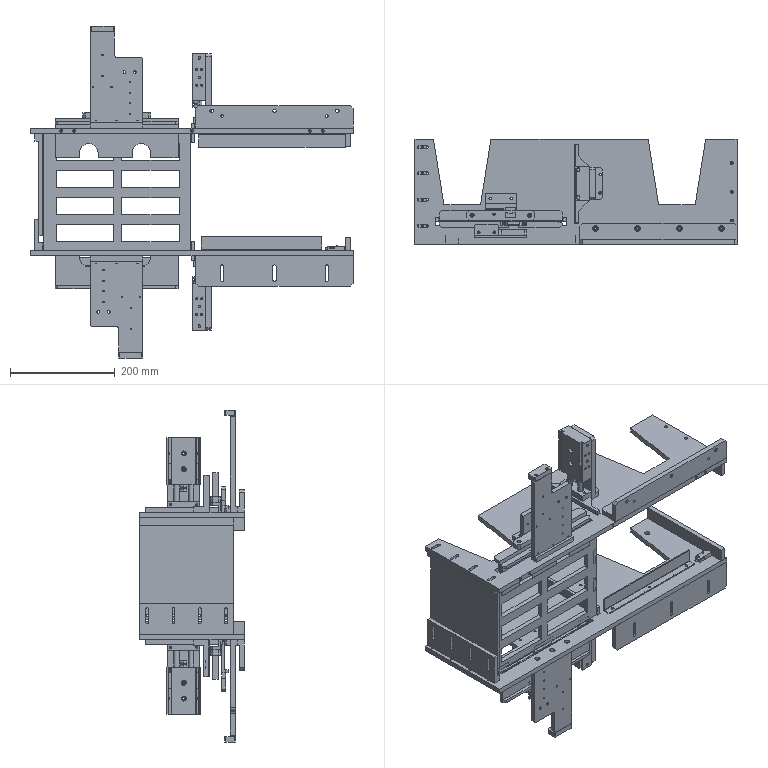Assembly | SolidWorks | mm | 36 component files | 36 solids | 1800 faces | box 615 x 200.5 x 634 mm | volume 4530078 mm3 | plane 894 | cylinder 645 | cone 164 | spline 97 | commonest cylinder face diameters 5.5 x100 4.2 x84 3.3 x48 3.24 x48 2.5 x42 6 x40 5 x38 4.5 x38
Bill of materials:
2011FeederTray | 1 |  | Flat rectangular grid-like frame plate with eight rectangular through-openings in a 2 x 4 arrangement, split by one central bar and three cross bars.
FPJ-D21 | 1 |  | Rectangular block with a large round bore near one end, a short cylindrical pin sticking out of one end face, a small low cylindrical boss on the top face, and a shallow elongated rectangular recess or slot on one side face. Two corners are chamfered in one view.
P-SLJ-001-001 | 2 | 45# | Straight solid rectangular bar with three evenly spaced small holes on one long narrow face.
P-SLJ-001-002 | 1 | SUS 304 | Long thin-walled angle profile with an L-shaped section, unequal legs and a rounded inside and outside bend. One leg has four evenly spaced round holes along its length.
P-SLJ-001-003 | 1 | SUS 304 | Long thin-walled angle profile with an L-shaped section and a rounded bend, similar to an angle bracket. One leg has three evenly spaced round holes.
P-SLJ-001-004 | 1 | 45# | Thick bar with an L-shaped (stepped) section: a tall upright web with a lower foot or ledge running along one side. The web has four evenly spaced elongated slots running vertically.
P-SLJ-001-005 | 1 | 45# | Thin, near-square plate with a thicker lip or step along one edge, giving an L-like section. There are four holes in the lip's top face and four holes near the opposite edge of the main face.
P-SLJ-001-006 | 1 | 45# | Thick angle bar with an L-shaped section and chamfered end corners. One leg has three elongated slots and the other leg has four round holes.
P-SLJ-001-007 | 1 | 45# | Thick angle bar with an L-shaped section and chamfered corners. One leg has four evenly spaced holes; the other leg has larger and smaller holes in a mixed pattern. There are small steps at the ends of one leg.
P-SLJ-001-008 | 1 | 45# | Large flat plate with two trapezoidal notches cut into one long edge. It has four short slots along one end, a long rectangular through-slot, a narrow perpendicular slot, and many small holes scattered across it.
P-SLJ-001-009 | 1 | A3 | Large flat plate with the same outline as unnamed part 1: two trapezoidal edge notches, four end slots, a long rectangular slot, a narrow slot, and many small holes. The small-hole pattern is slightly different, with some larger holes.
P-SLJ-002-001 | 2 | Al 6061 | Thin plate with a stepped outline: a rectangular upper region and a narrower lower tab, with filleted inside and outside corners and chamfered bottom corners. It has a thicker lip along the top edge with three holes, plus a pattern of small and medium holes through the face.
P-SLJ-002-002 | 2 | Al 6061 | T-shaped block: a long top bar sits on a narrower plate below it; the plate has four holes and chamfered lower corners.
P-SLJ-002-003 | 1 | A3 | Thin long plate with two round-bottomed U-slots cut in from one long edge. A thicker lip runs along the opposite edge, with a gap in the middle. The side view shows a tapered (beveled) edge.
SL-26 | 2 |  | Rectangular block with four chamfered vertical corners and two through holes near one long edge.
P-SLJ-003-001 | 1 | A3 | Thin long plate with two round-ended U-slots open to one long edge. A thicker lip with small holes and a central notch runs along the opposite edge. The edge opposite the lip is tapered.
P-SLJ-004-001 | 2 | A3 | L-shaped bracket: a tall upright plate on a short foot. The upright face has six holes and the foot has two holes.
P-SLJ-004-002 | 2 | A3 | Rectangular block with two through holes in its large face and a shallow rectangular slot across one end face.
P-SLJ-004-003 | 2 | A3 | Long flat bar with chamfered corners. It has two larger holes at the ends and three smaller holes near the middle, one of them off-center.
P-SLJ-004-004 | 2 | A3 | Long bar with an L-shaped section. Three legs hang down from it, one at each end and one in the middle, and each leg has a pointed or chamfered tip. The top has a row of holes.
body CXSM20-20-Z73 | 2 |  | Rectangular block with holes on several faces. There are two holes on the large face, a pattern of seven holes on a narrow side face, and small notches at the top edges.
rod CXSM20-20-Z73 | 2 |  | Rectangular base block with two upright cylindrical pins. There are vertical holes in the top face near each end and holes in a long side face.
P-SLJ-005-001 | 2 | A3 | L-shaped bracket: a tall plate with chamfered top corners and two small holes, on a short foot with two holes.
P-SLJ-005-002 | 2 | A3 | Angle-section bar. One leg is a full-length strip, and the other flange widens into a trapezoidal center section with two holes.
Mates:
1. distance | P-SLJ-001-008-1 face at (-76, 0, 1225.634) dir (0, 0, -1) | P-SLJ-001-009-2 face at (-76, 0, 1001.634) dir (0, 0, 1)
2. coincident | P-SLJ-001-009-2 face at (231.5, -100, 1001.634) dir (1, 0, 0) | P-SLJ-001-008-1 face at (231.5, -100, 1235.634) dir (1, 0, 0)
3. coincident | P-SLJ-001-009-2 face at (-383.5, -100, 1001.634) dir (0, -1, 0) | P-SLJ-001-008-1 face at (-383.5, -100, 1235.634) dir (0, -1, 0)
4. coincident | P-SLJ-001-007-2 face at (231.5, -100.5, 1235.634) dir (0, 0, -1) | P-SLJ-001-008-1 face at (-76, 0, 1235.634) dir (0, 0, 1)
5. concentric | P-SLJ-001-008-1 face at (221.5, 55, 1235.634) dir (0, 0, 1) r 2.75 | P-SLJ-001-001-1 face at (221.5, 55, 1225.634) dir (0, 0, 1) r 2.1
6. concentric | P-SLJ-001-008-1 face at (221.5, -55, 1235.634) dir (0, 0, 1) r 2.75 | P-SLJ-001-001-1 face at (221.5, -55, 1225.634) dir (0, 0, 1) r 2.1
7. coincident | P-SLJ-001-008-1 face at (-76, 0, 1225.634) dir (0, 0, -1) | P-SLJ-001-001-1 face at (221.5, 0, 1225.634) dir (0, 0, 1)
8. concentric | P-SLJ-001-007-2 face at (-38.5, -70, 1245.634) dir (0, 0, 1) r 5.5 | P-SLJ-001-008-1 face at (-38.5, -70, 1235.634) dir (0, 0, 1) r 2.5
9. concentric | P-SLJ-001-007-2 face at (201.5, -70, 1245.634) dir (0, 0, 1) r 5.5 | P-SLJ-001-008-1 face at (201.5, -70, 1235.634) dir (0, 0, 1) r 2.5
10. coincident | P-SLJ-001-008-1 face at (-76, 0, 1225.634) dir (0, 0, -1) | P-SLJ-001-002-1 face at (76.5, -65.5, 1225.634) dir (0, 0, 1)
11. coincident | P-SLJ-001-008-1 face at (-383.5, 100, 1235.634) dir (0, 1, 0) | P-SLJ-001-005-1 face at (-376, 100, 1225.634) dir (0, 1, 0)
12. coincident | P-SLJ-001-008-1 face at (-76, 0, 1225.634) dir (0, 0, -1) | P-SLJ-001-005-1 face at (-376, 100, 1225.634) dir (0, 0, 1)
13. distance | P-SLJ-001-005-1 face at (-376, 100, 1225.634) dir (-1, 0, 0) | P-SLJ-001-008-1 face at (-383.5, -100, 1235.634) dir (-1, 0, 0)
14. coincident | P-SLJ-001-009-2 face at (-76, 0, 1001.634) dir (0, 0, 1) | P-SLJ-001-003-2 face at (56.5, -65.5, 1001.634) dir (0, 0, -1)
15. concentric | P-SLJ-001-009-2 face at (221.5, 55, 1001.634) dir (0, 0, 1) r 2.75 | P-SLJ-001-001-2 face at (221.5, 55, 1001.634) dir (0, 0, -1) r 2.1
16. concentric | P-SLJ-001-009-2 face at (221.5, -55, 1001.634) dir (0, 0, 1) r 2.75 | P-SLJ-001-001-2 face at (221.5, -55, 1001.634) dir (0, 0, -1) r 2.1
17. coincident | P-SLJ-001-009-2 face at (-76, 0, 1001.634) dir (0, 0, 1) | P-SLJ-001-001-2 face at (221.5, 0, 1001.634) dir (0, 0, -1)
18. concentric | P-SLJ-001-009-2 face at (-38.5, -70, 1001.634) dir (0, 0, 1) r 2.5 | P-SLJ-001-006-3 face at (-38.5, -70, 981.634) dir (0, 0, -1) r 3.3
19. concentric | P-SLJ-001-009-2 face at (201.5, -70, 1001.634) dir (0, 0, 1) r 2.5 | P-SLJ-001-006-3 face at (201.5, -70, 981.634) dir (0, 0, -1) r 3.3
20. coincident | P-SLJ-001-009-2 face at (-76, 0, 991.634) dir (0, 0, -1) | P-SLJ-001-006-3 face at (-68.5, -100.5, 991.634) dir (0, 0, 1)
21. coincident | P-SLJ-001-005-1 face at (-376, 100, 1225.634) dir (0, 1, 0) | P-SLJ-001-004-1 face at (-368.5, 100, 1016.634) dir (0, 1, 0)
22. coincident | P-SLJ-001-009-2 face at (-76, 0, 1001.634) dir (0, 0, 1) | P-SLJ-001-004-1 face at (-376, 100, 1001.634) dir (0, 0, -1)
23. coincident | P-SLJ-001-005-1 face at (-368.5, 100, 1029.634) dir (-1, 0, 0) | P-SLJ-001-004-1 face at (-368.5, 100, 1061.634) dir (1, 0, 0)
24. coincident | P-SLJ-001-008-1 face at (-76, 0, 1235.634) dir (0, 0, 1) | P-SLJ-003-1/P-SLJ-002-001-1 face at (-270, -83, 1235.634) dir (0, 0, -1)
25. coincident | P-SLJ-001-008-1 face at (-76, 0, 1235.634) dir (0, 0, 1) | P-SLJ-004-3/P-SLJ-004-001-1 face at (-249.5, -33, 1235.634) dir (0, 0, -1)
26. concentric | P-SLJ-001-008-1 face at (-239.5, -13, 1235.634) dir (0, 0, 1) r 2.1 | P-SLJ-004-3/P-SLJ-004-001-1 face at (-239.5, -13, 1245.634) dir (0, 0, 1) r 2.75
27. concentric | P-SLJ-001-008-1 face at (-199.5, -13, 1235.634) dir (0, 0, 1) r 2.1 | P-SLJ-004-3/P-SLJ-004-001-1 face at (-199.5, -13, 1245.634) dir (0, 0, 1) r 2.75
28. coincident | P-SLJ-001-008-1 face at (-76, 0, 1235.634) dir (0, 0, 1) | P-SLJ-005-3/P-SLJ-005-001-1 face at (-49.5, -15.5, 1235.634) dir (0, 0, -1)
29. width | P-SLJ-005-3/P-SLJ-005-002-1 face at (-77.5, 89.5, 1243.634) dir (0, 1, 0) | P-SLJ-005-3/P-SLJ-005-002-1 face at (-77.5, -58.5, 1243.634) dir (0, -1, 0) | P-SLJ-001-008-1 face at (-70.5, -60, 1225.634) dir (0, 1, 0) | P-SLJ-001-008-1 face at (-70.5, 91, 1225.634) dir (0, -1, 0)
30. width | P-SLJ-001-008-1 face at (-78.5, -60, 1225.634) dir (1, 0, 0) | P-SLJ-001-008-1 face at (-70.5, -60, 1225.634) dir (-1, 0, 0) | P-SLJ-005-3/P-SLJ-005-002-1 face at (-77.5, 89.5, 1243.634) dir (-1, 0, 0) | P-SLJ-005-3/P-SLJ-005-002-1 face at (-71.5, 89.5, 1208.634) dir (1, 0, 0)
31. concentric | P-SLJ-001-009-2 face at (-29.5, 33, 1001.634) dir (0, 0, 1) r 2.1 | P-SLJ-005-4/P-SLJ-005-001-1 face at (-29.5, 33, 981.634) dir (0, 0, -1) r 2.75
32. concentric | P-SLJ-001-009-2 face at (-29.5, -2, 1001.634) dir (0, 0, 1) r 2.1 | P-SLJ-005-4/P-SLJ-005-001-1 face at (-29.5, -2, 981.634) dir (0, 0, -1) r 2.75
33. coincident | P-SLJ-001-009-2 face at (-76, 0, 991.634) dir (0, 0, -1) | P-SLJ-005-4/P-SLJ-005-001-1 face at (-49.5, 46.5, 991.634) dir (0, 0, 1)
34. coincident | P-SLJ-001-009-2 face at (-76, 0, 991.634) dir (0, 0, -1) | P-SLJ-002-2/P-SLJ-002-001-1 face at (-170, -83, 991.634) dir (0, 0, 1)
35. concentric | P-SLJ-001-009-2 face at (-199.5, -13, 1001.634) dir (0, 0, 1) r 2.1 | P-SLJ-004-4/P-SLJ-004-001-1 face at (-199.5, -13, 981.634) dir (0, 0, -1) r 2.75
36. concentric | P-SLJ-001-009-2 face at (-239.5, -13, 1001.634) dir (0, 0, 1) r 2.1 | P-SLJ-004-4/P-SLJ-004-001-1 face at (-239.5, -13, 981.634) dir (0, 0, -1) r 2.75
37. coincident | P-SLJ-001-009-2 face at (-76, 0, 991.634) dir (0, 0, -1) | P-SLJ-004-4/P-SLJ-004-001-1 face at (-189.5, -33, 991.634) dir (0, 0, 1)
38. concentric | P-SLJ-001-008-1 face at (121.5, -65.5, 1225.634) dir (0, 0, -1) r 1.65 | P-SLJ-001-002-1 face at (121.5, -65.5, 1223.634) dir (0, 0, -1) r 2.25
39. concentric | P-SLJ-001-008-1 face at (-58.5, -65.5, 1225.634) dir (0, 0, -1) r 1.65 | P-SLJ-001-002-1 face at (-58.5, -65.5, 1223.634) dir (0, 0, -1) r 2.25
40. concentric | P-SLJ-001-009-2 face at (156.5, -65.5, 1001.634) dir (0, 0, 1) r 1.65 | P-SLJ-001-003-2 face at (156.5, -65.5, 1003.634) dir (0, 0, 1) r 2.25
41. concentric | P-SLJ-001-009-2 face at (-43.5, -65.5, 1001.634) dir (0, 0, 1) r 1.65 | P-SLJ-001-003-2 face at (-43.5, -65.5, 1003.634) dir (0, 0, 1) r 2.25
42. concentric | P-SLJ-001-009-2 face at (186.5, -66, 1001.634) dir (0, 0, 1) r 1.25 | FPJ-D21-1 face at (186.5, -66, 1009.634) dir (0, 0, 1) r 3.25
43. coincident | P-SLJ-001-009-2 face at (-76, 0, 1001.634) dir (0, 0, 1) | FPJ-D21-1 face at (215.5, -74, 1001.634) dir (0, 0, -1)
44. concentric | P-SLJ-001-008-1 face at (-260, -80.5, 1225.634) dir (0, 0, -1) r 2.75 | P-SLJ-003-1/P-SLJ-002-001-1 face at (-260, -80.5, 1235.634) dir (0, 0, -1) r 2.1
45. concentric | P-SLJ-001-008-1 face at (-180, -80.5, 1225.634) dir (0, 0, -1) r 2.75 | P-SLJ-003-1/P-SLJ-002-001-1 face at (-180, -80.5, 1235.634) dir (0, 0, -1) r 2.1
46. coincident | P-SLJ-001-009-2 face at (-76, 0, 991.634) dir (0, 0, -1) | P-SLJ-002-2/P-SLJ-002-001-1 face at (-170, -83, 991.634) dir (0, 0, 1)
47. concentric | P-SLJ-001-009-2 face at (-260, -80.5, 1001.634) dir (0, 0, 1) r 2.75 | P-SLJ-002-2/P-SLJ-002-001-1 face at (-260, -80.5, 991.634) dir (0, 0, 1) r 2.1
48. concentric | P-SLJ-001-009-2 face at (-180, -80.5, 1001.634) dir (0, 0, 1) r 2.75 | P-SLJ-002-2/P-SLJ-002-001-1 face at (-180, -80.5, 991.634) dir (0, 0, 1) r 2.1
49. coincident | P-SLJ-002-2/P-SLJ-002-003-1 face at (-102.5, -57, 928.634) dir (0, 1, 0) | 2011FeederTray-1 face at (-78.25, -57, 1225.634) dir (0, -1, 0)
50. width | 2011FeederTray-1 face at (-78.25, -57, 1225.634) dir (0, 0, 1) | 2011FeederTray-1 face at (-78.25, -57, 1001.634) dir (0, 0, -1) | P-SLJ-001-009-2 face at (-76, 0, 1001.634) dir (0, 0, 1) | P-SLJ-001-008-1 face at (-76, 0, 1225.634) dir (0, 0, -1)
51. width | P-SLJ-005-3/P-SLJ-005-002-1 face at (-77.5, 89.5, 1243.634) dir (-1, 0, 0) | P-SLJ-001-005-1 face at (-361, 100, 1225.634) dir (1, 0, 0) | 2011FeederTray-1 face at (-78.25, -57, 1225.634) dir (1, 0, 0) | 2011FeederTray-1 face at (-360.25, -57, 1225.634) dir (-1, 0, 0)
52. coincident | P-SLJ-002-002-1 face at (63, 26, 0) dir (-1, 0, 0) | P-SLJ-002-003-1 face at (63, 14, 117.5) dir (1, 0, 0)
53. coincident | P-SLJ-002-001-1 face at (185, 0, 50) dir (1, 0, 0) | SL-26-1 face at (185, 0, 50) dir (-1, 0, 0)
54. concentric | P-SLJ-002-001-1 face at (185, 5, 12) dir (1, 0, 0) r 2.1 | SL-26-1 face at (195, 5, 12) dir (1, 0, 0) r 2.75
55. concentric | P-SLJ-002-001-1 face at (185, 5, 42) dir (1, 0, 0) r 2.1 | SL-26-1 face at (195, 5, 42) dir (1, 0, 0) r 2.75
56. coincident | P-SLJ-002-002-1 face at (63, 26, 0) dir (-1, 0, 0) | P-SLJ-003-001-1 face at (63, 14, 117.5) dir (1, 0, 0)
57. coincident | P-SLJ-002-001-1 face at (185, 0, 50) dir (1, 0, 0) | SL-26-1 face at (185, 0, 4) dir (-1, 0, 0)
58. concentric | P-SLJ-002-001-1 face at (185, 5, 42) dir (1, 0, 0) r 2.1 | SL-26-1 face at (185, 5, 42) dir (-1, 0, 0) r 2.75
59. concentric | P-SLJ-002-001-1 face at (185, 5, 12) dir (1, 0, 0) r 2.1 | SL-26-1 face at (185, 5, 12) dir (-1, 0, 0) r 2.75
60. concentric | P-SLJ-004-002-1 face at (29, -12, -23) dir (-1, 0, 0) r 1.65 | P-SLJ-004-003-1 face at (19, -12, -23) dir (-1, 0, 0) r 4
61. concentric | P-SLJ-004-002-1 face at (29, -12, -13) dir (-1, 0, 0) r 1.65 | P-SLJ-004-003-1 face at (19, -12, -13) dir (-1, 0, 0) r 4
62. coincident | P-SLJ-004-002-1 face at (29, -12, -18) dir (-1, 0, 0) | P-SLJ-004-003-1 face at (29, -22, 65) dir (1, 0, 0)
63. concentric | P-SLJ-004-003-1 face at (29, -12, 55) dir (1, 0, 0) r 2.25 | P-SLJ-004-004-1 face at (19, -12, 55) dir (1, 0, 0) r 1.65
64. concentric | P-SLJ-004-003-1 face at (29, -12, -55) dir (1, 0, 0) r 2.25 | P-SLJ-004-004-1 face at (19, -12, -55) dir (1, 0, 0) r 1.65
65. coincident | P-SLJ-004-003-1 face at (19, -22, 65) dir (-1, 0, 0) | P-SLJ-004-004-1 face at (19, -22, 117.5) dir (1, 0, 0)
66. concentric | CXSM20-20-Z73-1/body CXSM20-20-Z73-1 face at (112, 0, -25) dir (0, 0, 1) r 4.75 | P-SLJ-005-001-1 face at (112, 0, 0) dir (0, 0, -1) r 2.1
67. concentric | CXSM20-20-Z73-1/body CXSM20-20-Z73-1 face at (82, 0, -25) dir (0, 0, 1) r 4.75 | P-SLJ-005-001-1 face at (82, 0, 0) dir (0, 0, -1) r 2.1
68. coincident | CXSM20-20-Z73-1/body CXSM20-20-Z73-1 face at (142, -32, 0) dir (0, 0, 1) | P-SLJ-005-001-1 face at (0, 31, 0) dir (0, 0, -1)
69. concentric | CXSM20-20-Z73-1/rod CXSM20-20-Z73-1 face at (27.5, 25, -12.5) dir (1, 0, 0) r 2.065 | P-SLJ-005-002-1 face at (22, 25, -12.5) dir (-1, 0, 0) r 2.75
70. concentric | CXSM20-20-Z73-1/rod CXSM20-20-Z73-1 face at (27.5, -25, -12.5) dir (1, 0, 0) r 2.065 | P-SLJ-005-002-1 face at (22, -25, -12.5) dir (-1, 0, 0) r 2.75
71. coincident | CXSM20-20-Z73-1/rod CXSM20-20-Z73-1 face at (28, 0, 0) dir (-1, 0, 0) | P-SLJ-005-002-1 face at (28, -74, -28) dir (1, 0, 0)
72. distance | rod CXSM20-20-Z73-1 face at (0, 0, 24) dir (0, 0, 1) | body CXSM20-20-Z73-1 face at (0, 0, 0) dir (0, 0, 1)
73. concentric | body CXSM20-20-Z73-1 face at (14, 12.5, -22) dir (0, 0, 1) r 5.1 | rod CXSM20-20-Z73-1 face at (14, 12.5, -22) dir (0, 0, 1) r 5
74. concentric | body CXSM20-20-Z73-1 face at (-14, 12.5, -22) dir (0, 0, 1) r 5.1 | rod CXSM20-20-Z73-1 face at (-14, 12.5, -22) dir (0, 0, 1) r 5